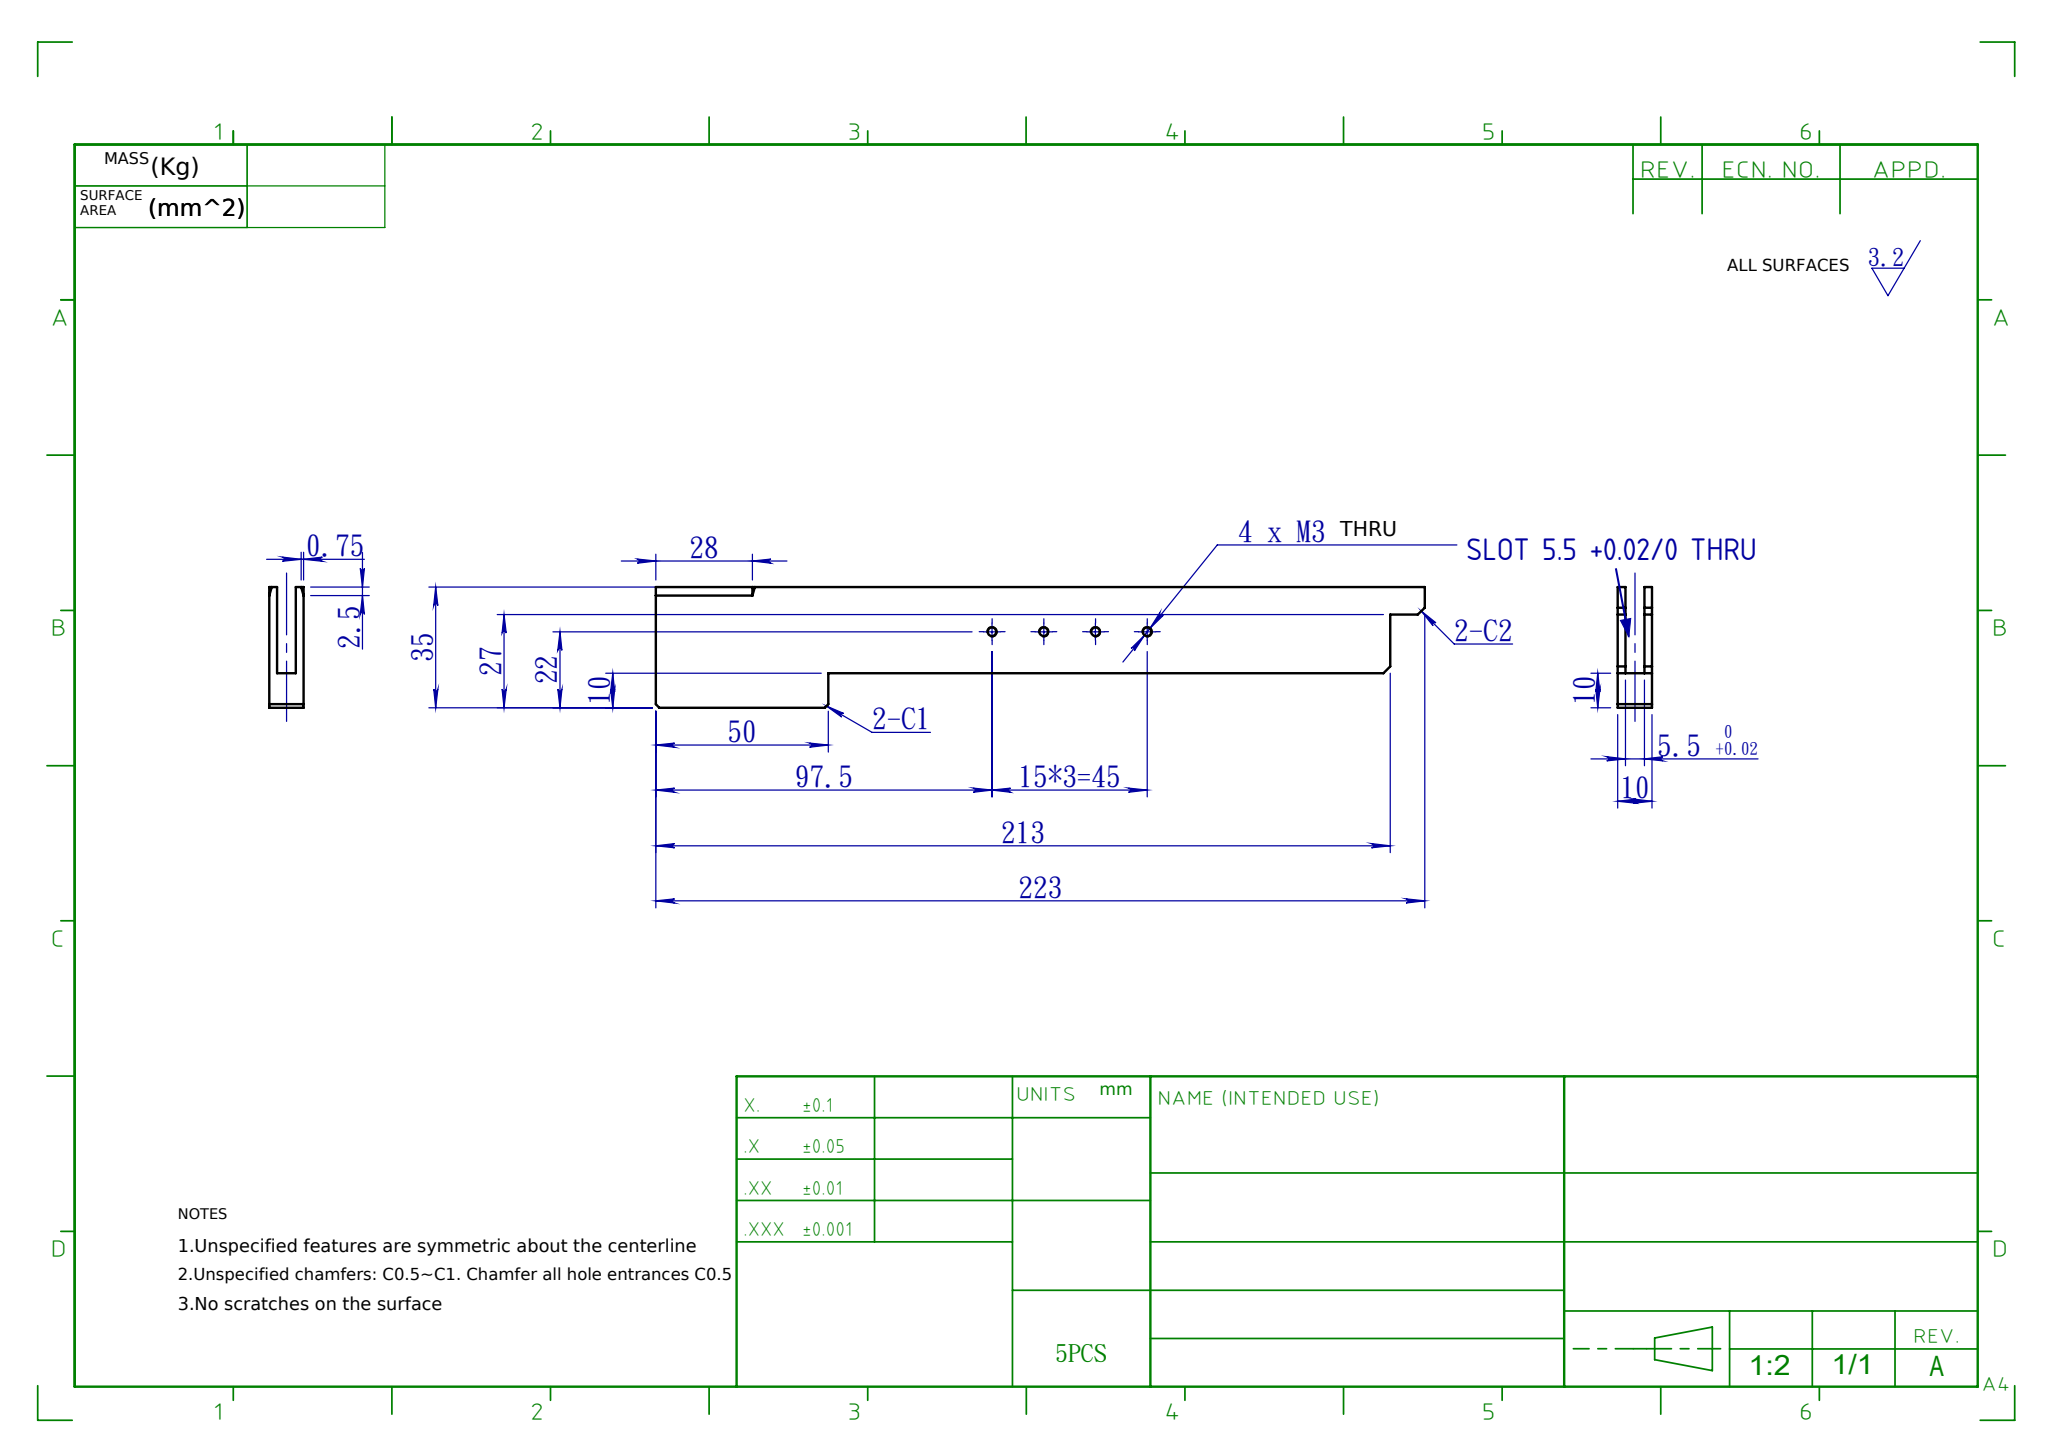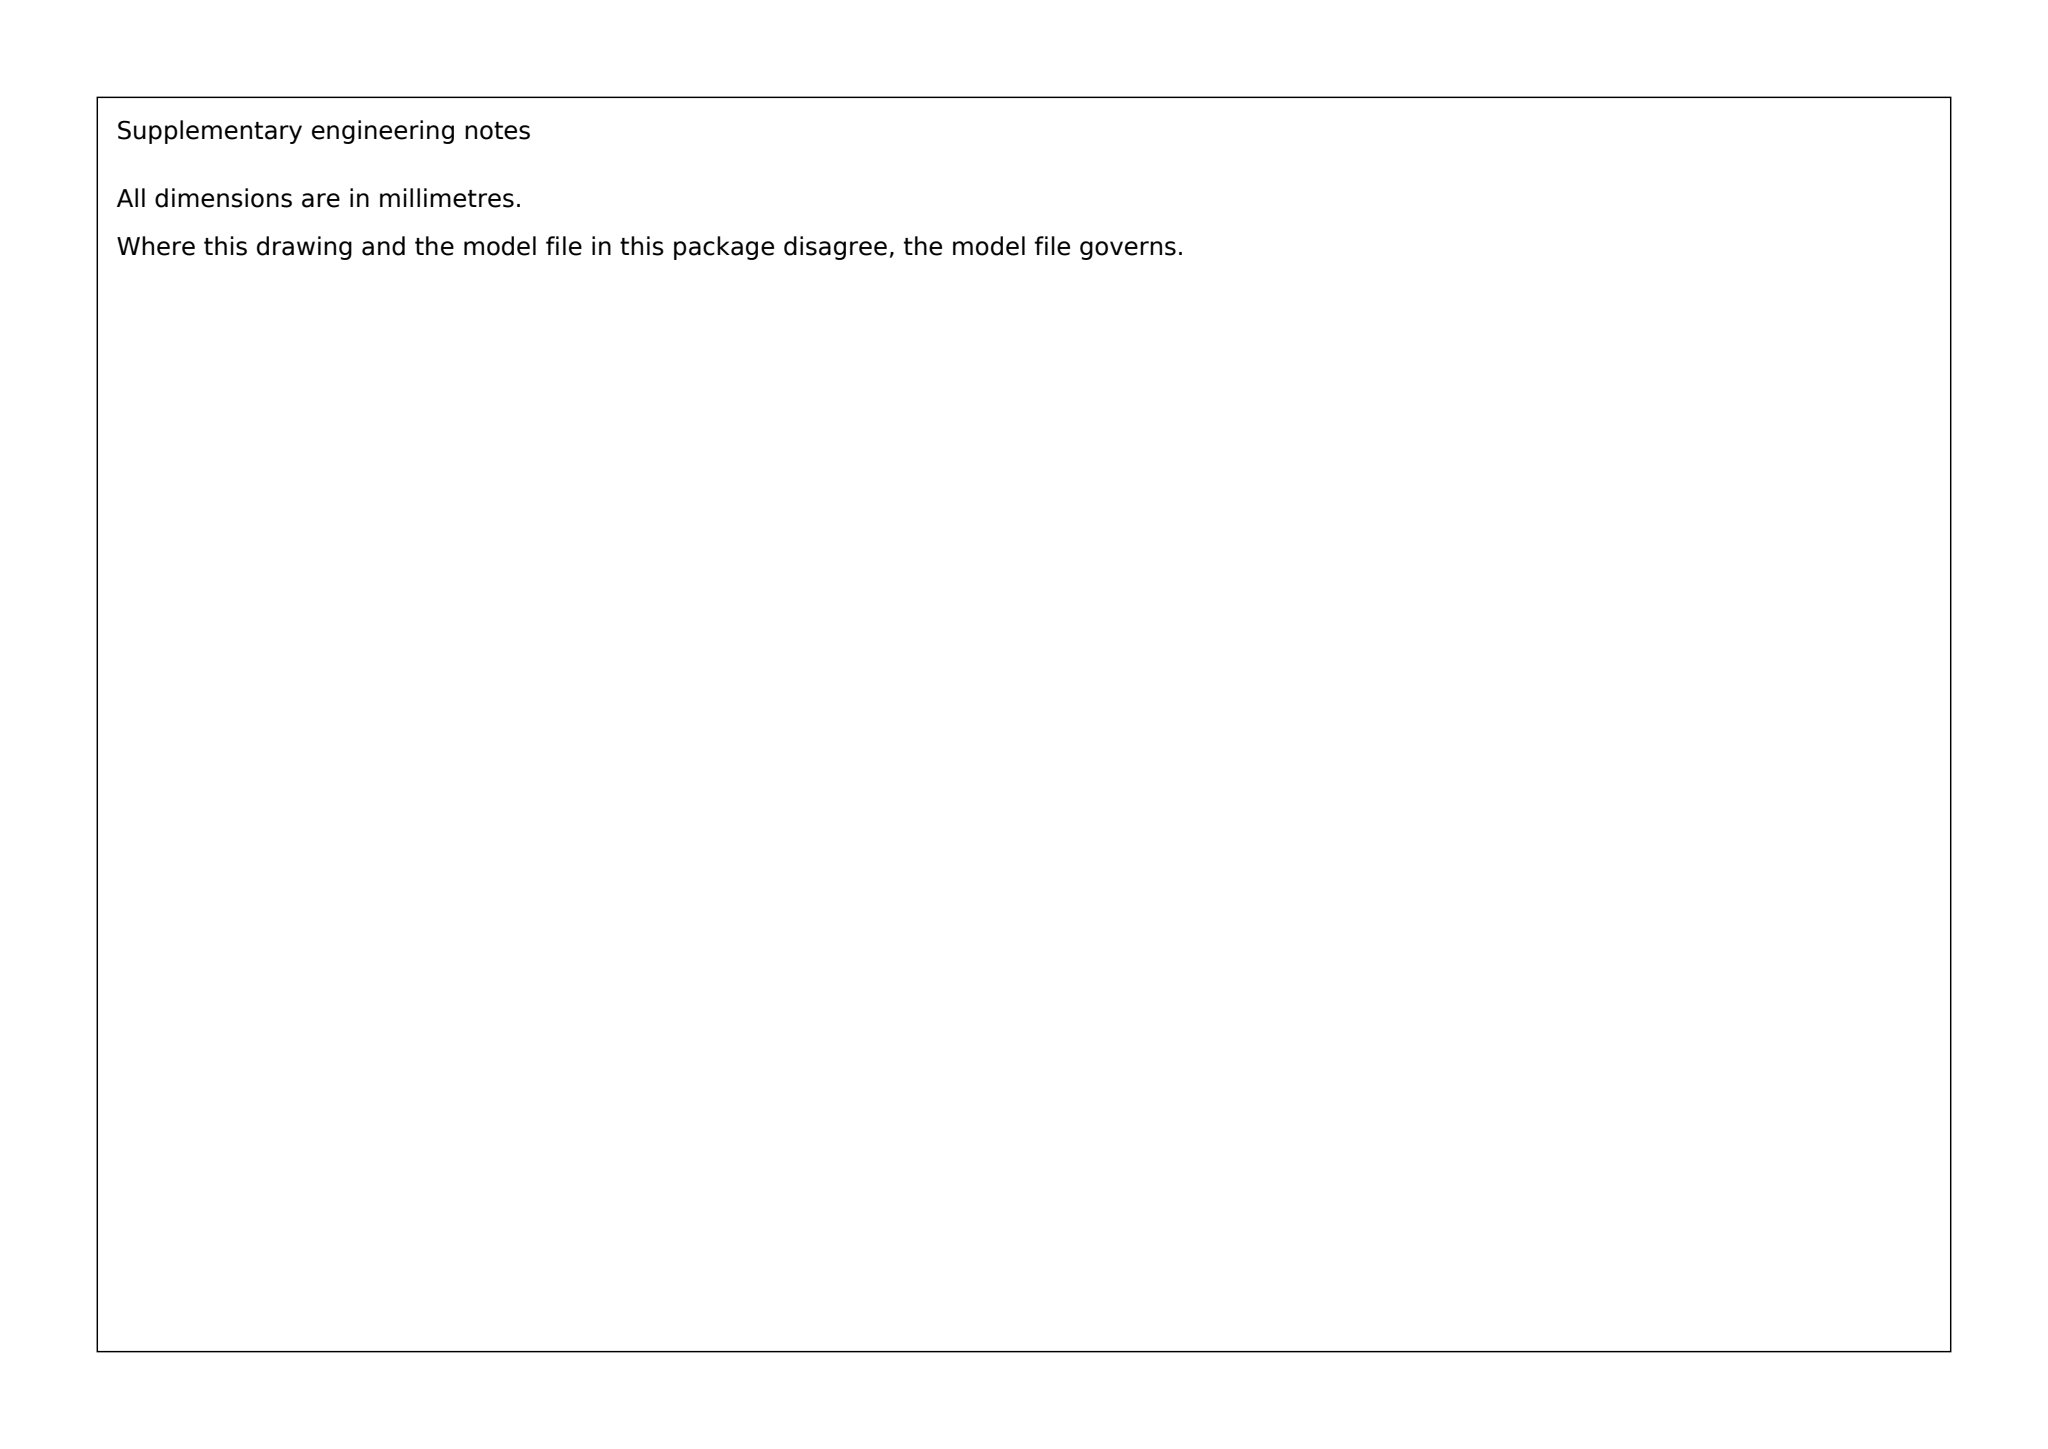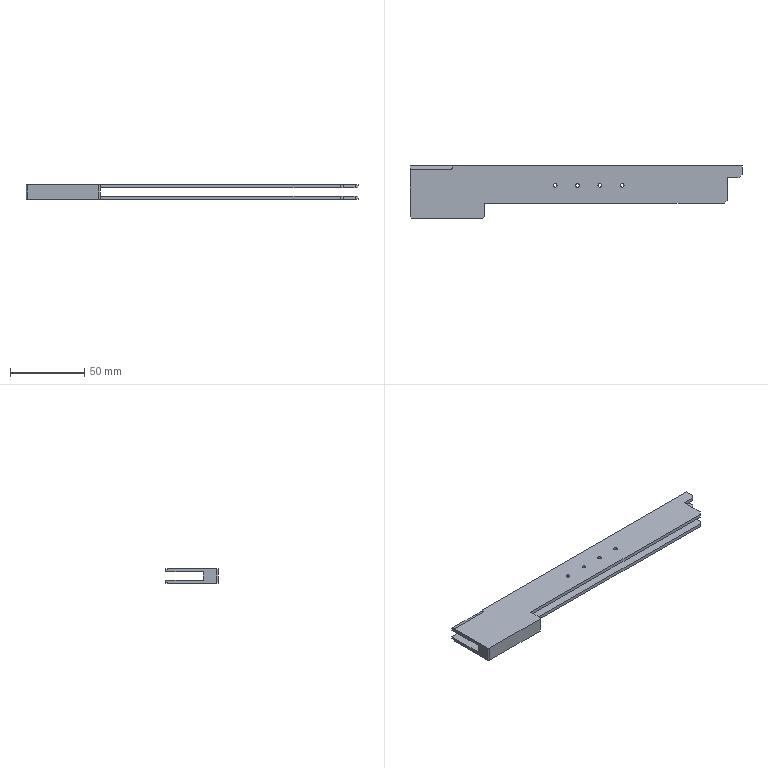Part | SolidWorks | mm | 1 solid | 44 faces | box 223 x 35 x 10 mm | volume 29153 mm3 | plane 28 | cylinder 16 | commonest cylinder face diameters 2.5 x16
Drawing notes:
SLOT WIDTH 5.5 +0.02/0 THRU, 2.3 FROM EACH FACE | from the solid: z-planes at 2.3 and 7.8 over y 10-35 give slot width 5.5; part thk 10